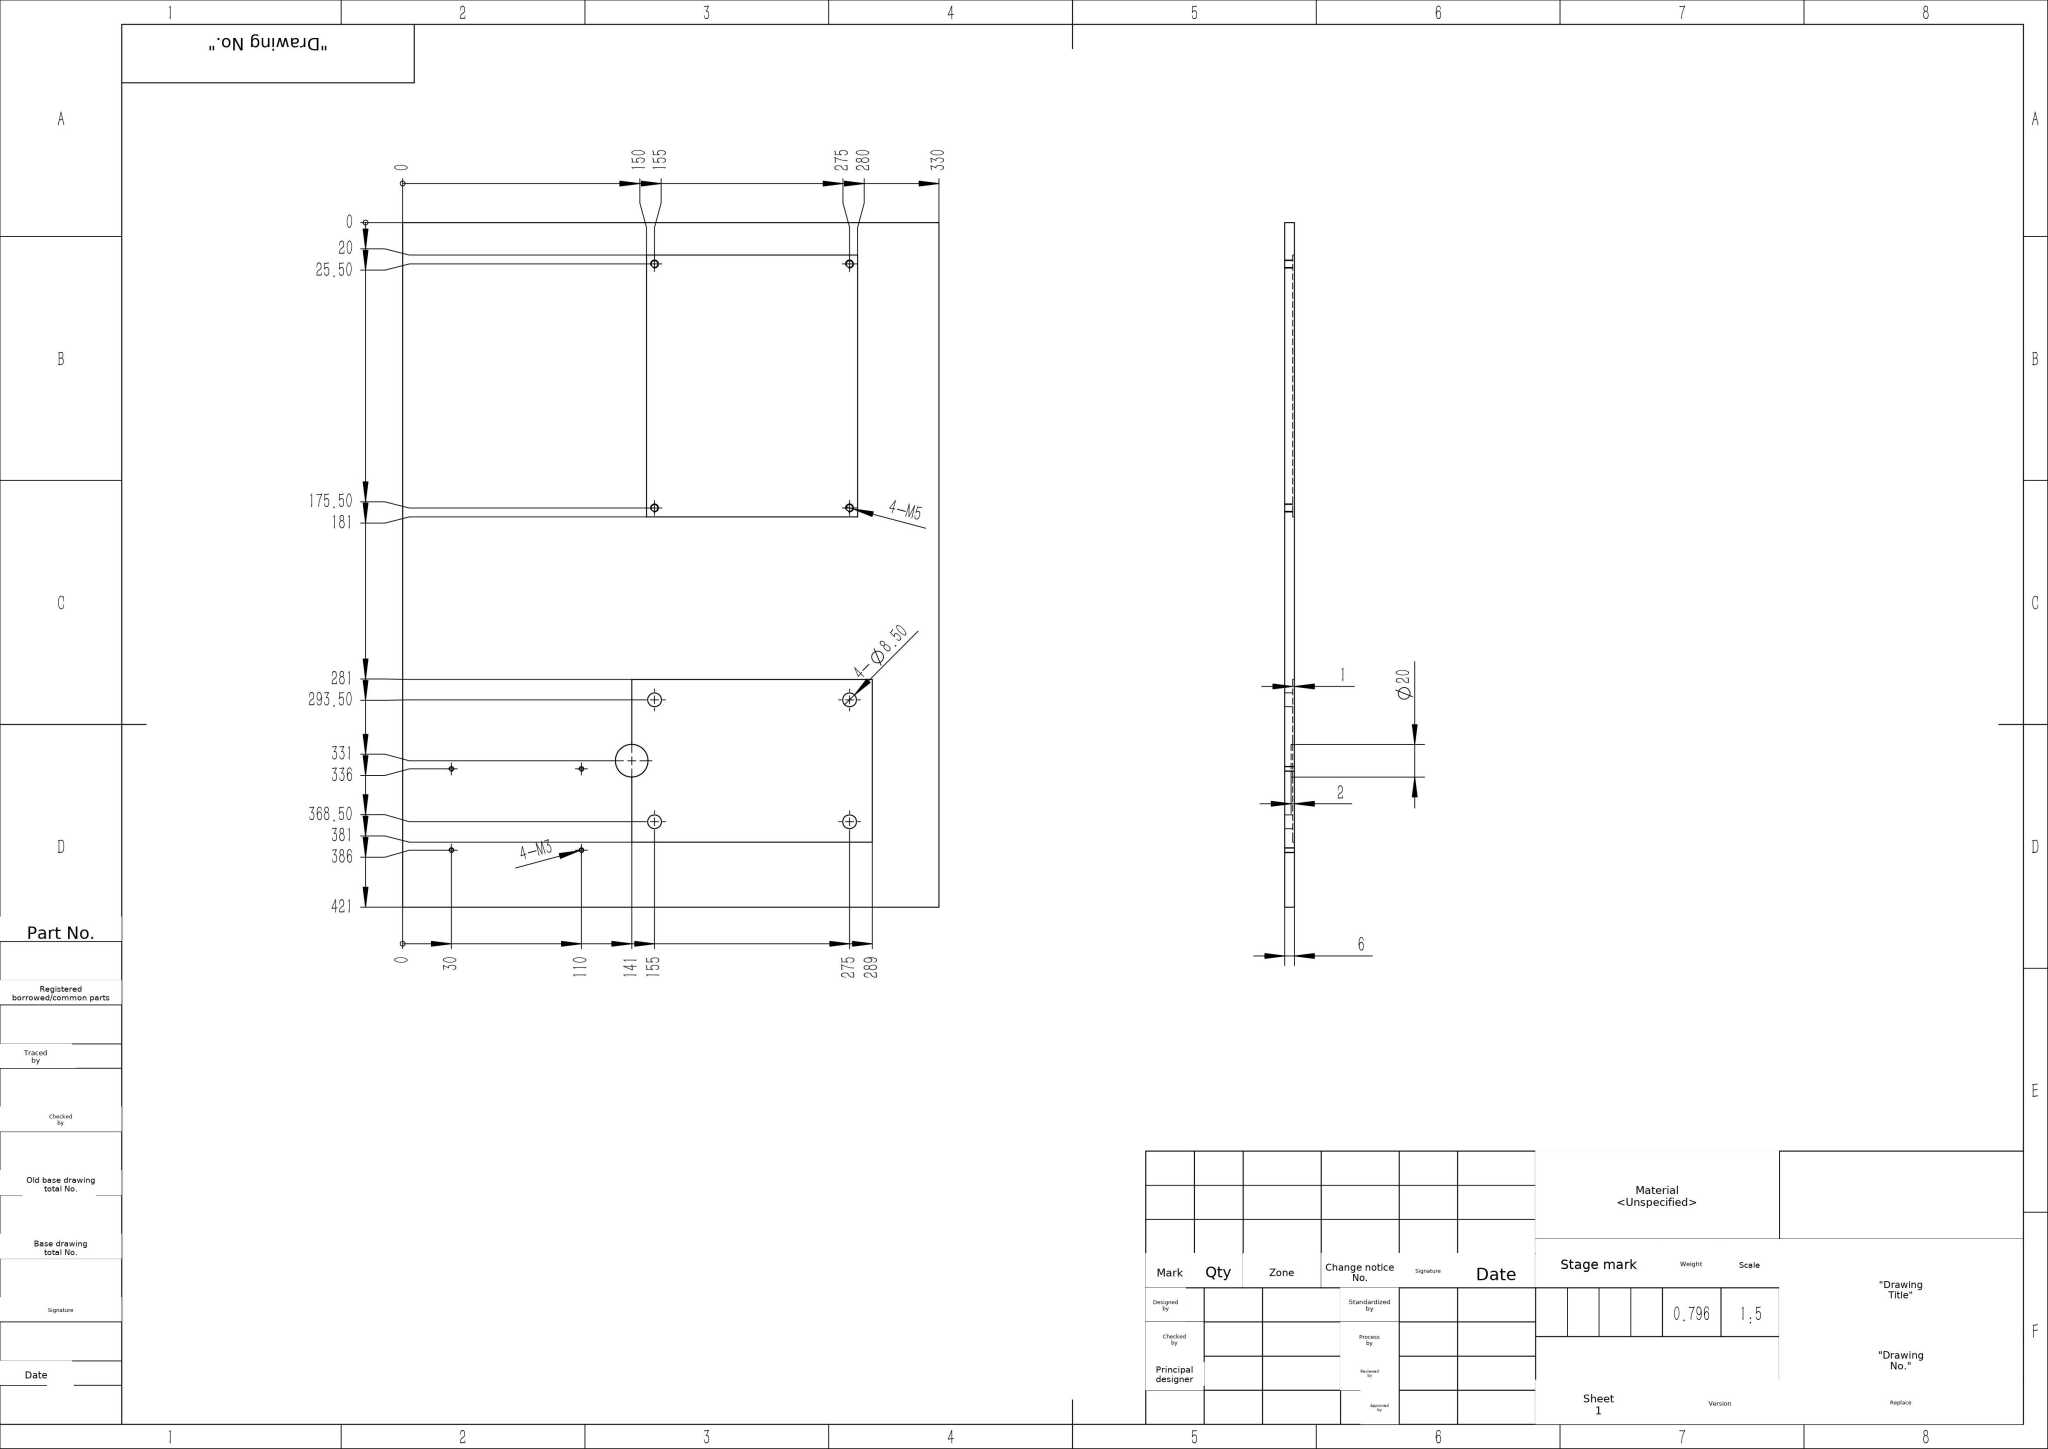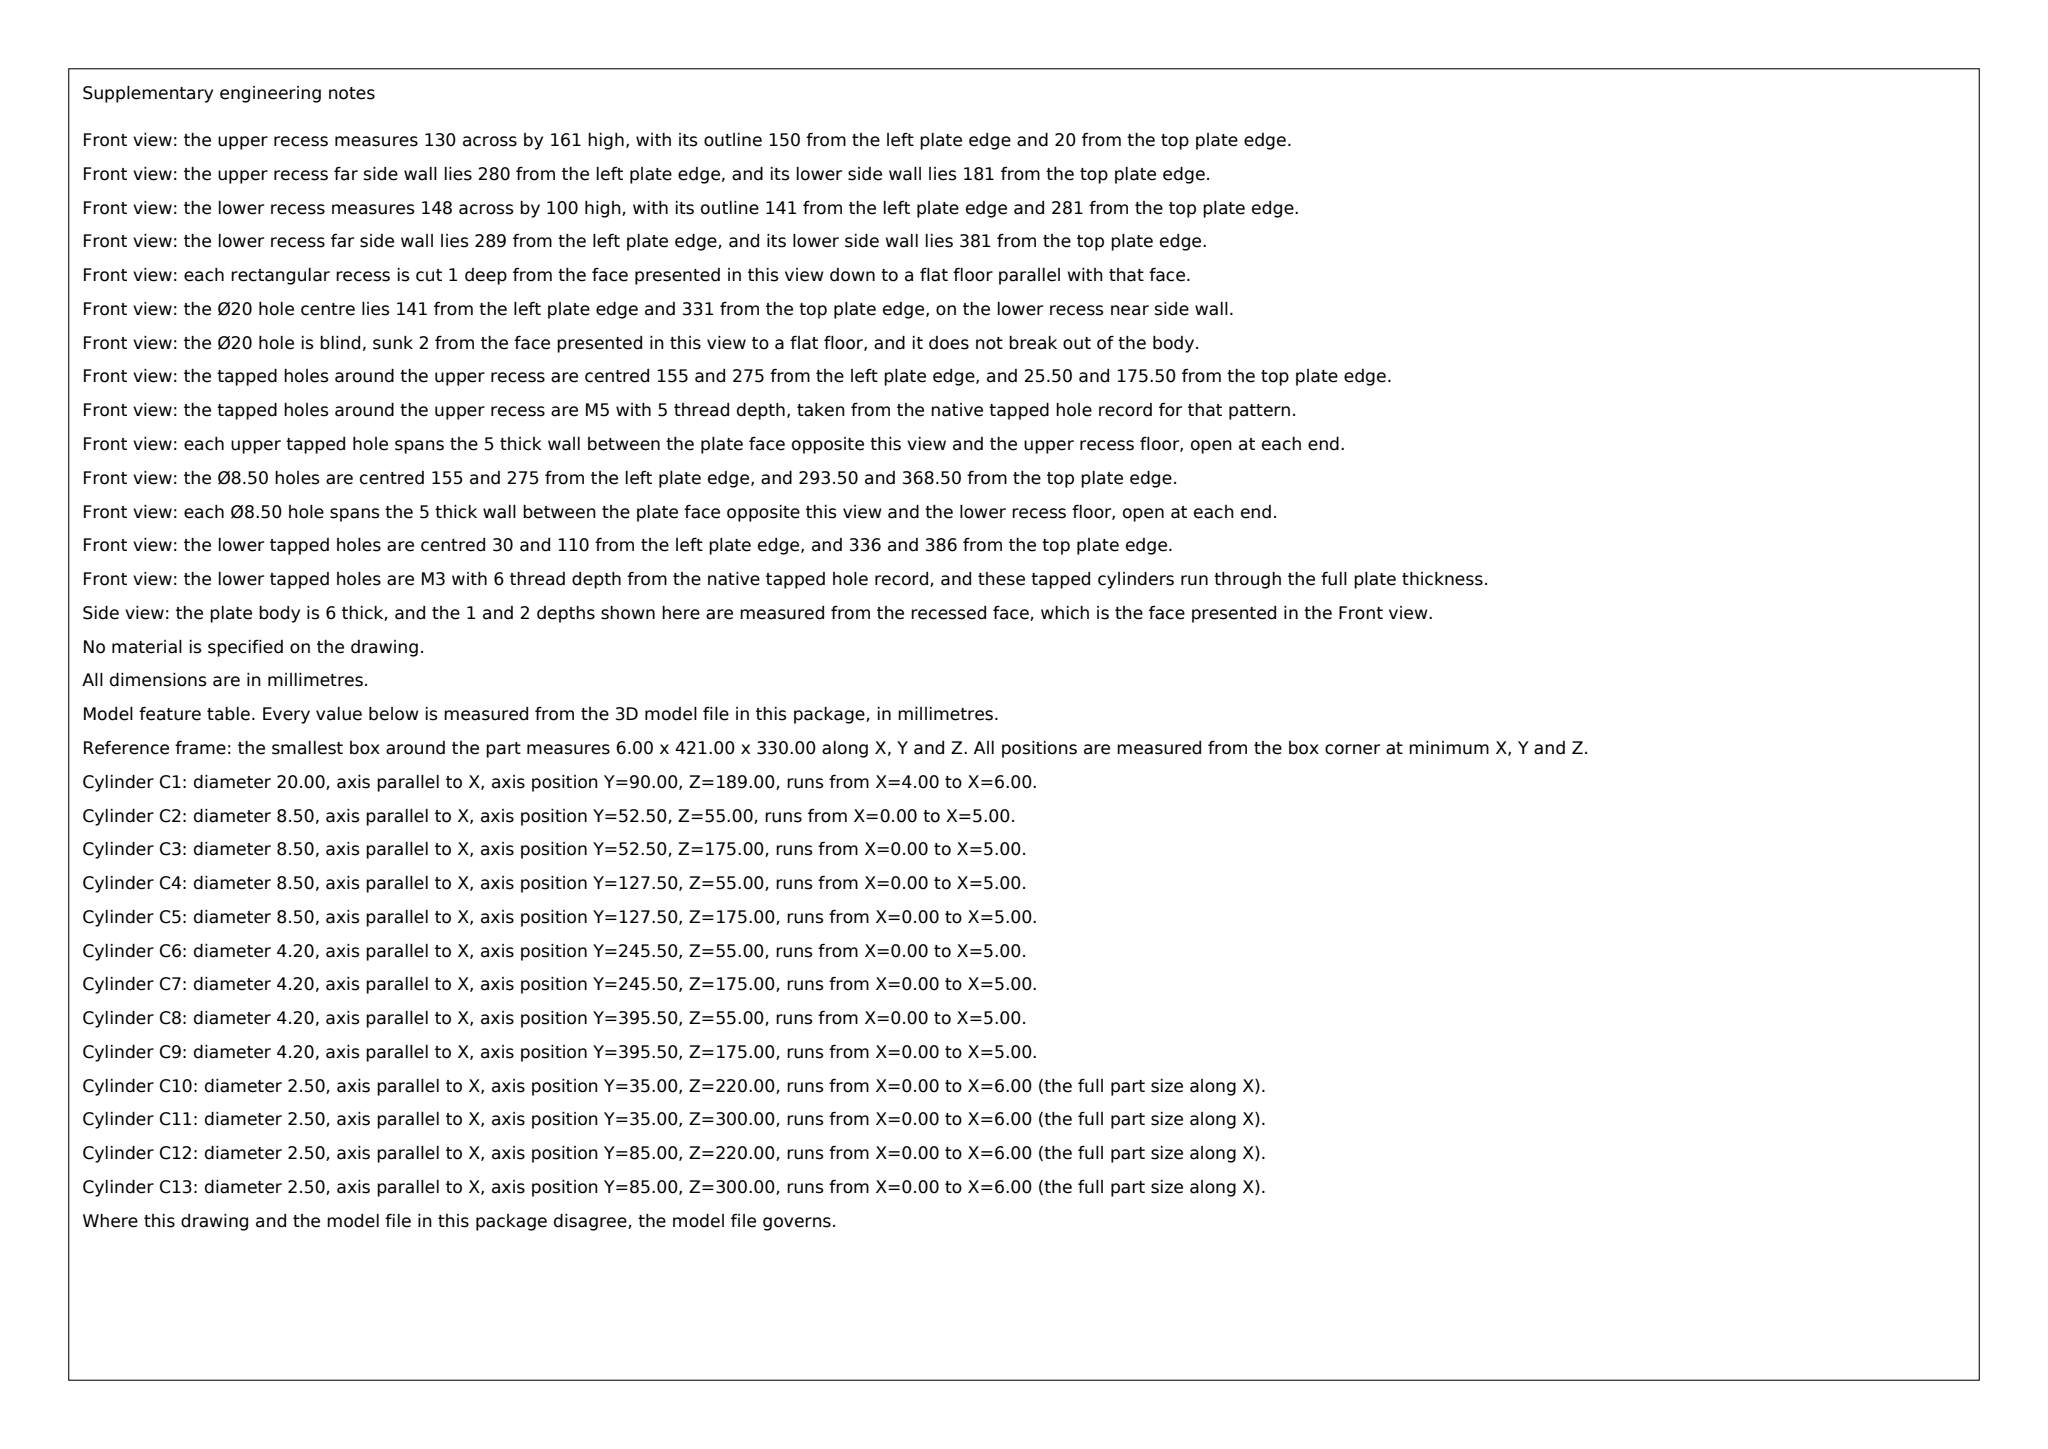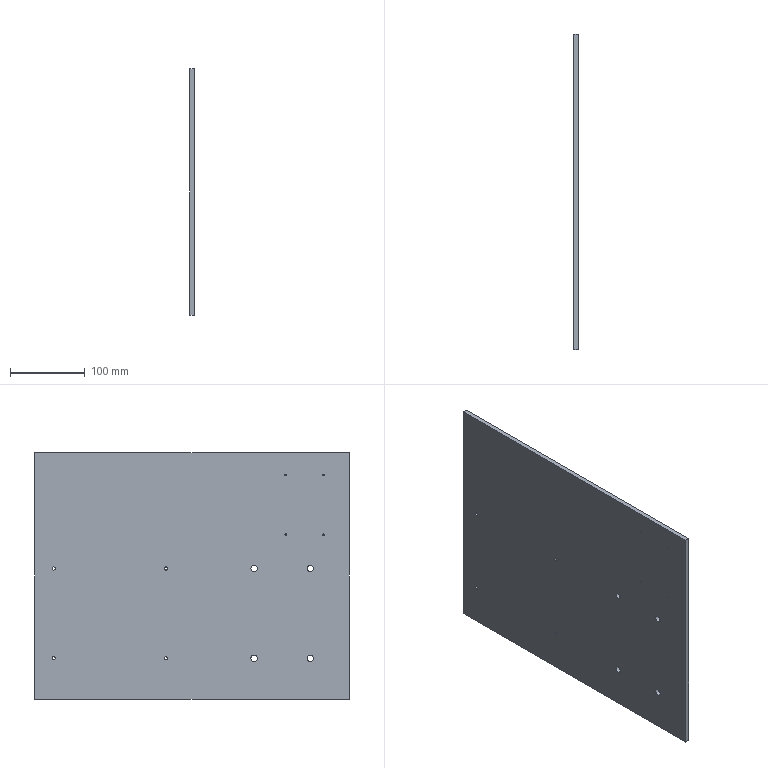Part | SolidWorks | mm | 1 solid | 44 faces | box 6 x 421 x 330 mm | volume 795849 mm3 | cylinder 26 | plane 18 | commonest cylinder face diameters 2.5 x8 8.5 x8 4.2 x8 20 x2
Drawing notes:
RECESS 150-280 X 20-181: DP 1 FROM BACK FACE | from the solid: z planes 50 & 180 (330-z = 150/280), y planes 240 & 401 (421-y = 20/181), floor plane x=5 vs face x=6 → 1 deep
RECESS 141-289 X 281-381: DP 1 FROM BACK FACE | from the solid: z planes 41 & 189 (330-z = 141/289), y planes 40 & 140 (421-y = 281/381), 2nd floor plane x=5 vs face x=6 → 1 deep
Ø20 DP 2 FROM BACK FACE, SAME SIDE AS RECESSES | from the solid: cylinder dia 20, axis x, length 2, pos y=90 (421-90=331), z=189 (330-189=141); floor plane x=4 vs face x=6
PLATE THK 6; ALL POCKETS MACHINED INTO BACK FACE | from the solid: bbox x = 6.0; planes x=0 and x=6 outer faces; recess floors x=5 (2X), Ø20 floor x=4
build123d program:
from build123d import *

# Parameters (mm, degrees)
SKETCH1_W                 = 330
SKETCH1_H                 = 421
BOSS_EXTRUDE1_DEPTH       = 6
SKETCH2_W                 = 130
SKETCH2_H                 = 161
SKETCH2_W_2               = 148
SKETCH2_H_2               = 100
CUT_EXTRUDE1_DEPTH        = 1
M5_TAPPED_HOLE1_D         = 4.2
SIZE_MM_DOWEL_PIN_HOLE1_D = 8.5
SKETCH8_R                 = 10
CUT_EXTRUDE2_DEPTH        = 2
M3_TAPPED_HOLE1_D         = 2.5


with BuildPart() as part:
    # Sketch1 → Boss-Extrude1 (new body)
    with BuildSketch(Plane(origin=(0, 0, 0), x_dir=(0, 0, -1), z_dir=(1, 0, 0))):
        Rectangle(SKETCH1_W, SKETCH1_H)
    extrude(amount=BOSS_EXTRUDE1_DEPTH)

    # Sketch2 → Cut-Extrude1 (cut)
    with BuildSketch(Plane(origin=(6, 0, 0), x_dir=(0, 0, -1), z_dir=(1, 0, 0))):
        with Locations((50, 110)):
            Rectangle(SKETCH2_W, SKETCH2_H)
        with Locations((50, -120.5)):
            Rectangle(SKETCH2_W_2, SKETCH2_H_2)
    extrude(amount=-CUT_EXTRUDE1_DEPTH, mode=Mode.SUBTRACT)

    # M5 Tapped Hole1 (through all)
    with Locations(Plane(origin=(5, 0, 0), x_dir=(0, 0, -1), z_dir=(1, 0, 0))):
        with Locations((-10, 185), (-10, 35), (110, 35), (110, 185)):
            Hole(M5_TAPPED_HOLE1_D / 2)

    # Size mm Dowel Pin Hole1 (through all)
    with Locations(Plane(origin=(5, 0, 0), x_dir=(0, 0, -1), z_dir=(1, 0, 0))):
        with Locations((-10, -83), (110, -83), (110, -158), (-10, -158)):
            Hole(SIZE_MM_DOWEL_PIN_HOLE1_D / 2)

    # Sketch8 → Cut-Extrude2 (cut)
    with BuildSketch(Plane(origin=(6, 0, 0), x_dir=(0, 0, -1), z_dir=(1, 0, 0))):
        with Locations((-24, -120.5)):
            Circle(SKETCH8_R)
    extrude(amount=-CUT_EXTRUDE2_DEPTH, mode=Mode.SUBTRACT)

    # M3 Tapped Hole1 (through all)
    with Locations(Plane(origin=(6, 0, 0), x_dir=(0, 0, -1), z_dir=(1, 0, 0))):
        with Locations((-135, -125.5), (-55, -125.5), (-135, -175.5), (-55, -175.5)):
            Hole(M3_TAPPED_HOLE1_D / 2)


solid = part.part